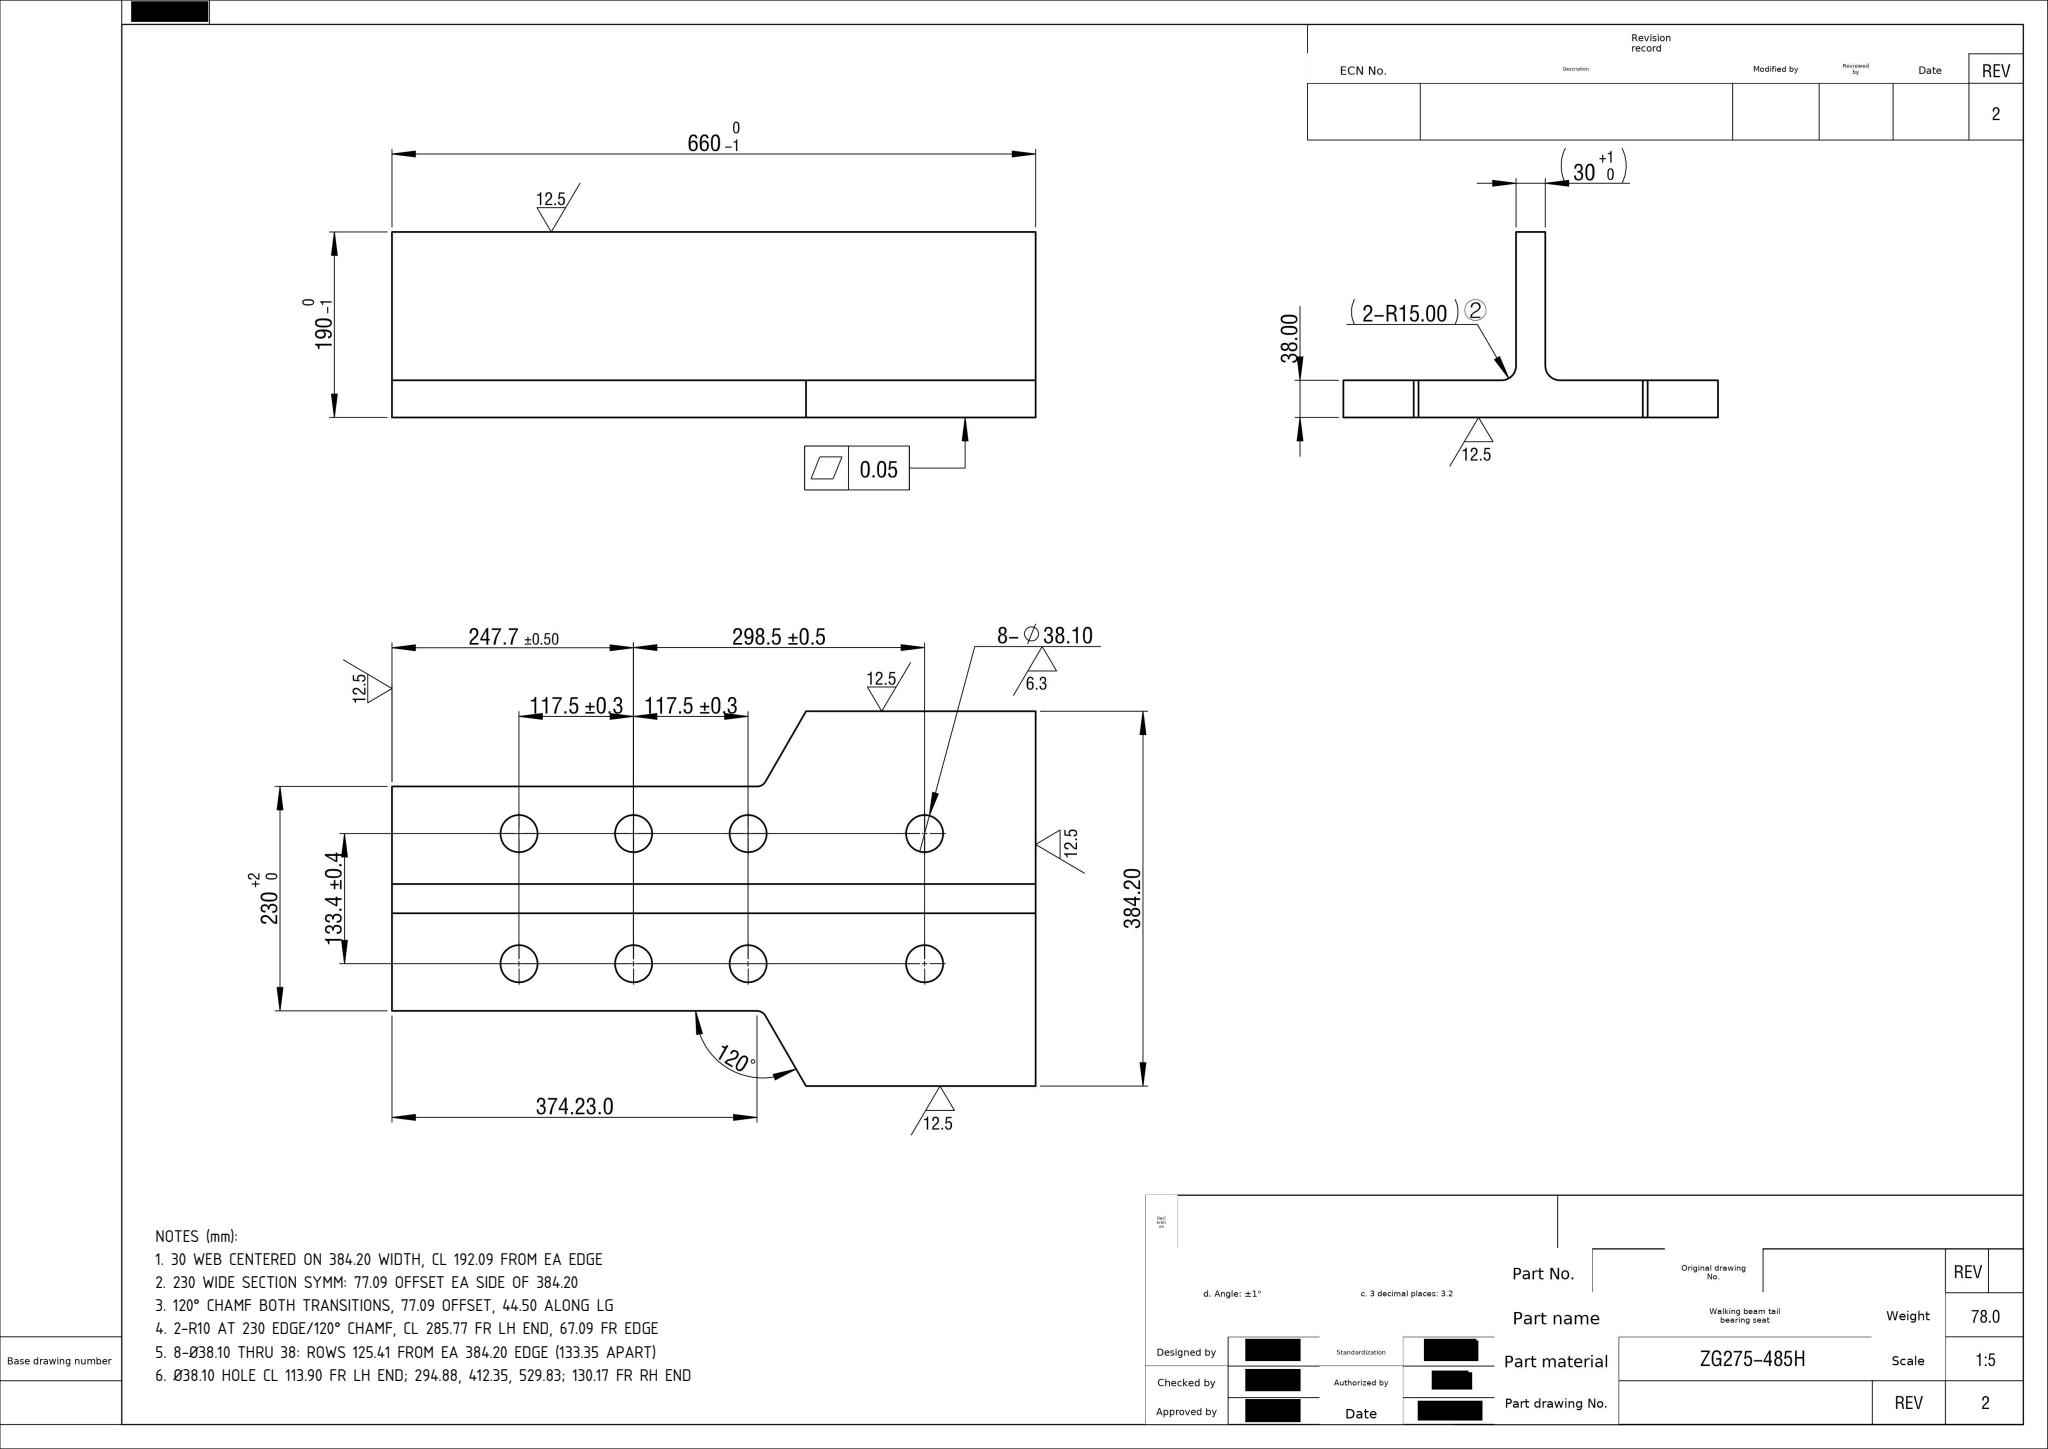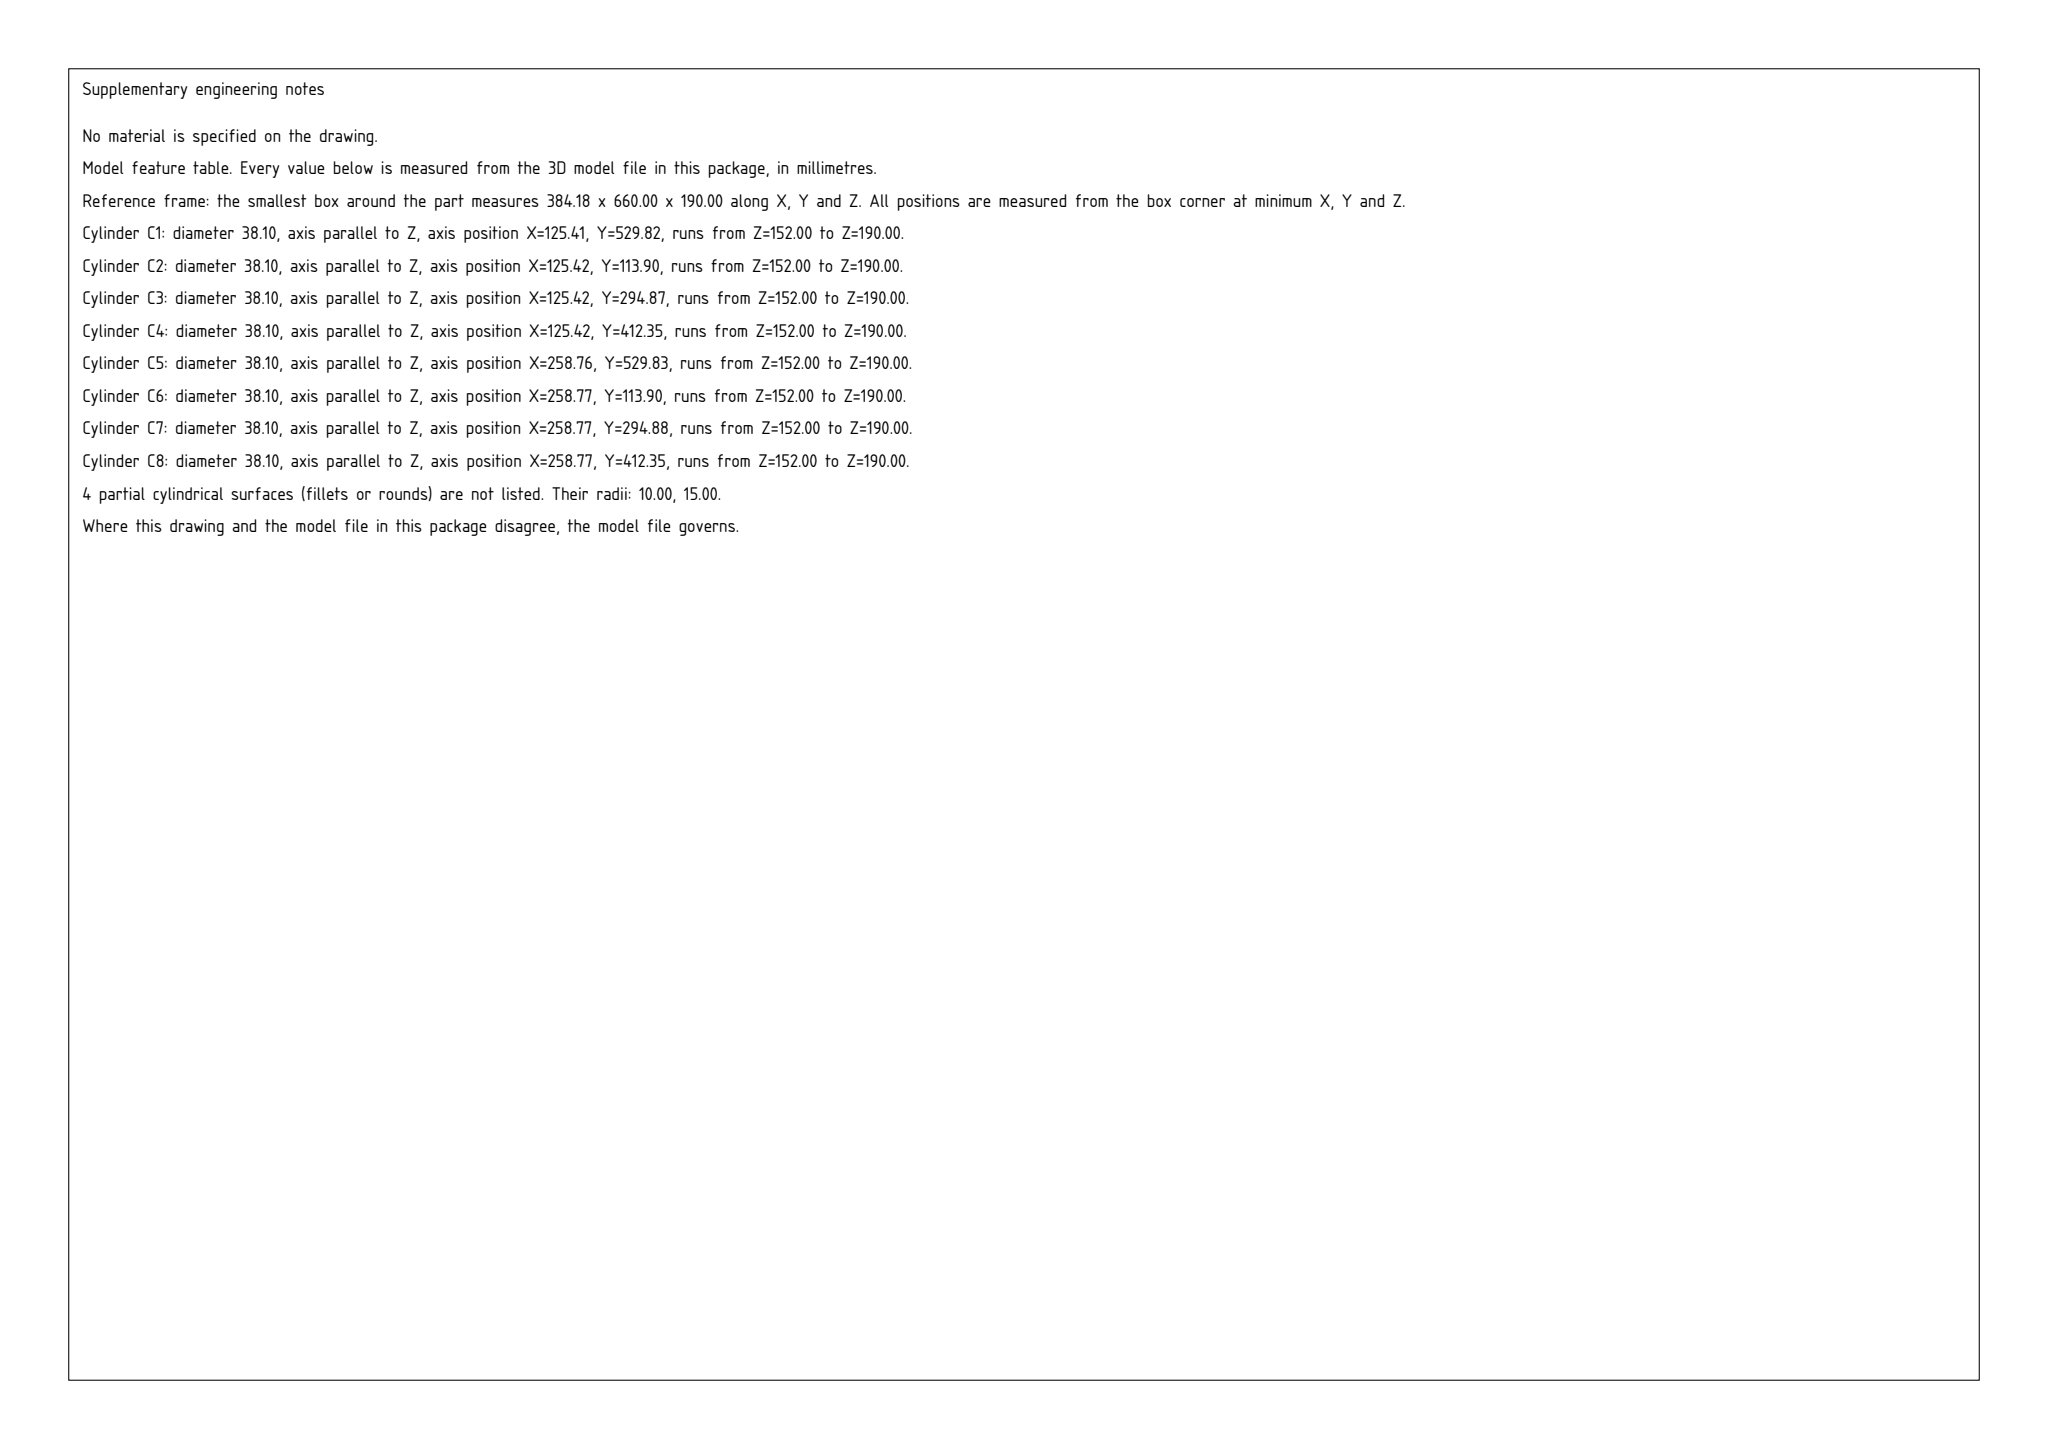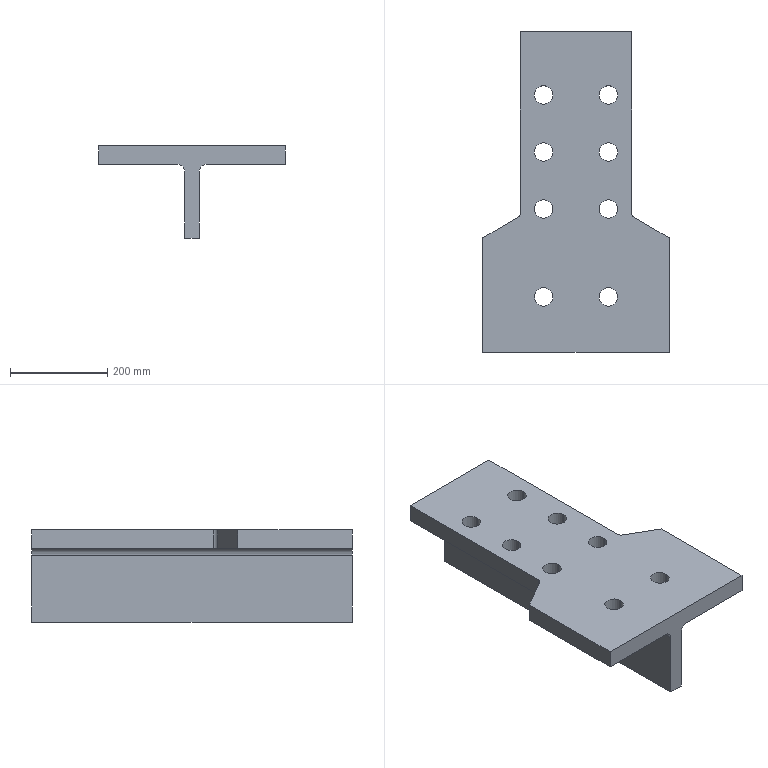Part | SolidWorks | mm | 1 solid | 34 faces | box 384.18 x 660 x 190 mm | volume 10005605 mm3 | cylinder 20 | plane 14 | commonest cylinder face diameters 38.1 x16 30 x2 20 x2
Drawing notes:
30 WEB CENTERED ON 384.20 WIDTH, CL 192.09 FROM EA EDGE | from the solid: x-planes 177.09 & 207.09 (30 thk); bbox x=384.175, CL 192.09
230 WIDE SECTION SYMM: 77.09 OFFSET EA SIDE OF 384.20 | from the solid: x-planes 77.09 & 307.09; (384.175-230)/2=77.09
120° CHAMF BOTH TRANSITIONS, 77.09 OFFSET, 44.50 ALONG LG | from the solid: 230 to 384.20 width; 77.09/tan60=44.50
2-R10 AT 230 EDGE/120° CHAMF, CL 285.77 FR LH END, 67.09 FR EDGE | from the solid: Ø20 z-cyls at (67.09,285.77) & (317.09,285.77), len 38
8-Ø38.10 THRU 38: ROWS 125.41 FROM EA 384.20 EDGE (133.35 APART) | from the solid: Ø38.1 z-cyls at x=125.41 & 258.76; 384.175-258.76=125.415
Ø38.10 HOLE CL 113.90 FR LH END; 294.88, 412.35, 529.83; 130.17 FR RH END | from the solid: hole y=113.90, 294.88, 412.35, 529.83; bbox y=660.0
build123d program:
from build123d import *

# Parameters (mm, degrees)
EXTRUDE1_DEPTH      = 252.65
EXTRUDE1_DEPTH_BACK = 417.35
FILLET1_R           = 15
CUT_EXTRUDE1_DEPTH  = 503.201
FILLET2_R           = 10
SKETCH5_W           = 404.175
SKETCH5_H           = 680
SKETCH5_W_2         = 384.175
SKETCH5_H_2         = 660
CUT_EXTRUDE4_DEPTH  = 503.201
SKETCH3_R           = 19.05
CUT_EXTRUDE2_DEPTH  = 481.578
SKETCH4_W           = 30
SKETCH4_H           = 3
SKETCH4_W_2         = 384.175
SKETCH4_H_2         = 7
CUT_EXTRUDE3_DEPTH  = 440


with BuildPart() as part:
    # Sketch1 → Extrude1 (new, two sides: drawn at the far end of the back side and taken through both)
    with BuildSketch(Plane(origin=(0, 0, 0), x_dir=(1, 0, 0), z_dir=(0, 1, 0)).offset(-EXTRUDE1_DEPTH_BACK)):
        Polygon((-195, 0), (-195, 38), (-15, 38), (-15, 193), (15, 193), (15, 38), (195, 38), (195, 0), (195, -7), (-195, -7), align=None)
    extrude(amount=EXTRUDE1_DEPTH + EXTRUDE1_DEPTH_BACK)

    # Fillet1
    fillet1_edges = [part.edges().sort_by_distance(p)[0] for p in [
        (-15, -82.35, -38),
        (15, -82.35, -38),
    ]]
    fillet(fillet1_edges, radius=FILLET1_R)

    # Sketch2 → Cut-Extrude1 (cut, through all)
    with BuildSketch(Plane.XY.offset(7)):
        Polygon((-195, 252.65), (-115, 252.65), (-115, -132.35), (-195, -178.538), align=None)
        Polygon((195, -178.538), (195, 252.65), (115, 252.65), (115, -132.35), align=None)
    extrude(amount=-CUT_EXTRUDE1_DEPTH, mode=Mode.SUBTRACT)

    # Fillet2
    fillet2_edges = [part.edges().sort_by_distance(p)[0] for p in [
        (-115, -132.35, -15.5),
        (115, -132.35, -15.5),
    ]]
    fillet(fillet2_edges, radius=FILLET2_R)

    # Sketch5 → Cut-Extrude4 (cut, through all)
    with BuildSketch(Plane.XY.offset(7)):
        with Locations((0, -82.35)):
            Rectangle(SKETCH5_W, SKETCH5_H)
        with Locations((0, -82.35)):
            Rectangle(SKETCH5_W_2, SKETCH5_H_2, mode=Mode.SUBTRACT)
    extrude(amount=-CUT_EXTRUDE4_DEPTH, mode=Mode.SUBTRACT)

    # Sketch3 → Cut-Extrude2 (cut, through all)
    with BuildSketch(Plane.XY.offset(-38)):
        with Locations(Location((-66.675, 117.475, 0), (0, 0, 180))):
            Circle(SKETCH3_R)
        with Locations(Location((-66.675, 0, 0), (0, 0, 180))):
            Circle(SKETCH3_R)
        with Locations(Location((-66.675, -117.475, 0), (0, 0, 180))):
            Circle(SKETCH3_R)
        with Locations(Location((-66.675, -298.45, 0), (0, 0, 180))):
            Circle(SKETCH3_R)
        with Locations(Location((66.675, -298.45, 0), (0, 0, 180))):
            Circle(SKETCH3_R)
        with Locations(Location((66.675, -117.475, 0), (0, 0, 180))):
            Circle(SKETCH3_R)
        with Locations(Location((66.675, 0, 0), (0, 0, 180))):
            Circle(SKETCH3_R)
        with Locations(Location((66.675, 117.475, 0), (0, 0, 180))):
            Circle(SKETCH3_R)
    extrude(amount=CUT_EXTRUDE2_DEPTH, mode=Mode.SUBTRACT)

    # Sketch4 → Cut-Extrude3 (cut, symmetric)
    with BuildSketch(Plane(origin=(0, 0, 0), x_dir=(1, 0, 0), z_dir=(0, 1, 0))):
        with Locations((0, 191.5)):
            Rectangle(SKETCH4_W, SKETCH4_H)
        with Locations((0, -3.5)):
            Rectangle(SKETCH4_W_2, SKETCH4_H_2)
    extrude(amount=CUT_EXTRUDE3_DEPTH, both=True, mode=Mode.SUBTRACT)


solid = part.part